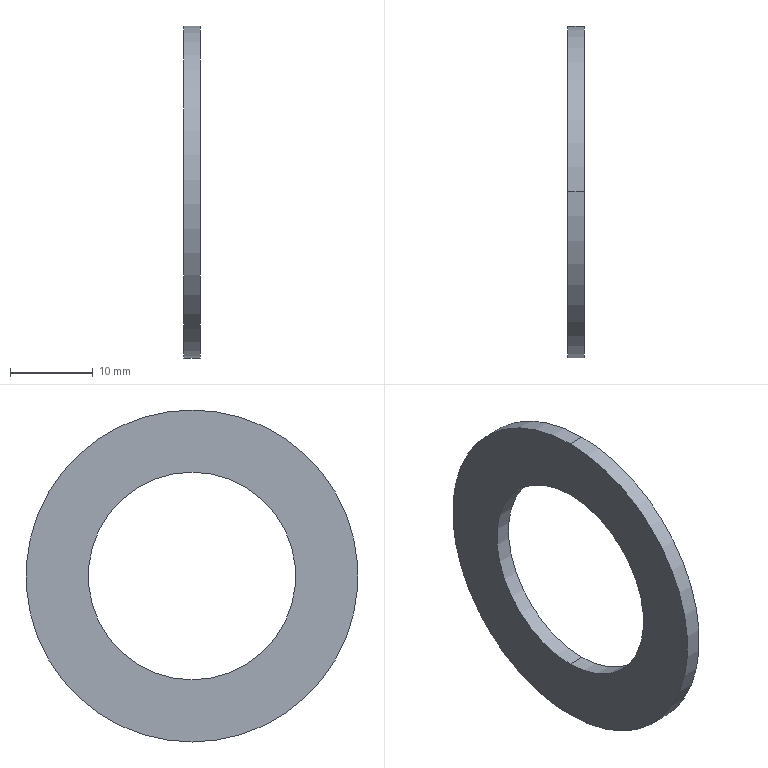Component | SolidWorks | 4-12-12ClampingAxisAssembly-1_4-12-8ClampingAxis51205BearingShim-1 | 1 solid | 6 faces | box 2 x 40 x 40 mm | volume 1532 mm3 | cylinder 4 | plane 2 | commonest cylinder face diameters 25 x2 40 x2
build123d program:
from build123d import *

# Parameters (mm, degrees)
SKETCH1_R      = 20
SKETCH1_R_2    = 12.5
EXTRUDE1_DEPTH = 2


with BuildPart() as part:
    # Sketch1 → Extrude1 (new body)
    with BuildSketch(Plane(origin=(0, 0, 0), x_dir=(1, 0, 0), z_dir=(0, 1, 0))):
        with Locations(Location((0, 0, 0), (0, 0, 270))):
            Circle(SKETCH1_R)
        with Locations(Location((0, 0, 0), (0, 0, 270))):
            Circle(SKETCH1_R_2, mode=Mode.SUBTRACT)
    extrude(amount=EXTRUDE1_DEPTH)


solid = part.part

# Placed as in the assembly
solid = solid.moved(Location((-53.809, -4.181, 0), (0, 0, 90)))
STEP:
#1=CARTESIAN_POINT('',(-2.197,-0.1646,-0.4921));
#2=VERTEX_POINT('',#1);
#3=CARTESIAN_POINT('',(-2.197,-0.1646,0.4921));
#4=VERTEX_POINT('',#3);
#5=CARTESIAN_POINT('',(-2.197,-0.1646,0.));
#6=DIRECTION('',(-1.,-0.,-0.));
#7=DIRECTION('',(0.,0.,1.));
#8=AXIS2_PLACEMENT_3D('',#5,#6,#7);
#9=CIRCLE('',#8,0.4921);
#10=EDGE_CURVE('',#2,#4,#9,.T.);
#11=ORIENTED_EDGE('',*,*,#10,.T.);
#12=CARTESIAN_POINT('',(-2.118,-0.1646,0.4921));
#13=VERTEX_POINT('',#12);
#14=CARTESIAN_POINT('',(-2.197,-0.1646,0.4921));
#15=DIRECTION('',(1.,0.,0.));
#16=VECTOR('',#15,39.37);
#17=LINE('',#14,#16);
#18=EDGE_CURVE('',#4,#13,#17,.T.);
#19=ORIENTED_EDGE('',*,*,#18,.T.);
#20=CARTESIAN_POINT('',(-2.118,-0.1646,-0.4921));
#21=VERTEX_POINT('',#20);
#22=CARTESIAN_POINT('',(-2.118,-0.1646,0.));
#23=DIRECTION('',(-1.,-0.,-0.));
#24=DIRECTION('',(0.,0.,1.));
#25=AXIS2_PLACEMENT_3D('',#22,#23,#24);
#26=CIRCLE('',#25,0.4921);
#27=EDGE_CURVE('',#21,#13,#26,.T.);
#28=ORIENTED_EDGE('',*,*,#27,.F.);
#29=CARTESIAN_POINT('',(-2.197,-0.1646,-0.4921));
#30=DIRECTION('',(1.,0.,0.));
#31=VECTOR('',#30,39.37);
#32=LINE('',#29,#31);
#33=EDGE_CURVE('',#2,#21,#32,.T.);
#34=ORIENTED_EDGE('',*,*,#33,.F.);
#35=EDGE_LOOP('',(#11,#19,#28,#34));
#36=FACE_OUTER_BOUND('',#35,.T.);
#37=CARTESIAN_POINT('',(-2.197,-0.1646,0.));
#38=DIRECTION('',(1.,0.,0.));
#39=DIRECTION('',(0.,-0.,-1.));
#40=AXIS2_PLACEMENT_3D('',#37,#38,#39);
#41=CYLINDRICAL_SURFACE('',#40,0.4921);
#42=ADVANCED_FACE('',(#36),#41,.F.);
#43=CARTESIAN_POINT('',(-2.197,-0.1646,0.7874));
#44=VERTEX_POINT('',#43);
#45=CARTESIAN_POINT('',(-2.197,-0.1646,-0.7874));
#46=VERTEX_POINT('',#45);
#47=CARTESIAN_POINT('',(-2.197,-0.1646,0.));
#48=DIRECTION('',(-1.,-0.,-0.));
#49=DIRECTION('',(0.,0.,1.));
#50=AXIS2_PLACEMENT_3D('',#47,#48,#49);
#51=CIRCLE('',#50,0.7874);
#52=EDGE_CURVE('',#44,#46,#51,.T.);
#53=ORIENTED_EDGE('',*,*,#52,.F.);
#54=CARTESIAN_POINT('',(-2.118,-0.1646,0.7874));
#55=VERTEX_POINT('',#54);
#56=CARTESIAN_POINT('',(-2.197,-0.1646,0.7874));
#57=DIRECTION('',(1.,0.,0.));
#58=VECTOR('',#57,39.37);
#59=LINE('',#56,#58);
#60=EDGE_CURVE('',#44,#55,#59,.T.);
#61=ORIENTED_EDGE('',*,*,#60,.T.);
#62=CARTESIAN_POINT('',(-2.118,-0.1646,-0.7874));
#63=VERTEX_POINT('',#62);
#64=CARTESIAN_POINT('',(-2.118,-0.1646,0.));
#65=DIRECTION('',(-1.,-0.,-0.));
#66=DIRECTION('',(0.,0.,1.));
#67=AXIS2_PLACEMENT_3D('',#64,#65,#66);
#68=CIRCLE('',#67,0.7874);
#69=EDGE_CURVE('',#55,#63,#68,.T.);
#70=ORIENTED_EDGE('',*,*,#69,.T.);
#71=CARTESIAN_POINT('',(-2.197,-0.1646,-0.7874));
#72=DIRECTION('',(1.,0.,0.));
#73=VECTOR('',#72,39.37);
#74=LINE('',#71,#73);
#75=EDGE_CURVE('',#46,#63,#74,.T.);
#76=ORIENTED_EDGE('',*,*,#75,.F.);
#77=EDGE_LOOP('',(#53,#61,#70,#76));
#78=FACE_OUTER_BOUND('',#77,.T.);
#79=CARTESIAN_POINT('',(-2.197,-0.1646,0.));
#80=DIRECTION('',(1.,0.,0.));
#81=DIRECTION('',(0.,-0.,-1.));
#82=AXIS2_PLACEMENT_3D('',#79,#80,#81);
#83=CYLINDRICAL_SURFACE('',#82,0.7874);
#84=ADVANCED_FACE('',(#78),#83,.T.);
#85=CARTESIAN_POINT('',(-2.197,-0.1646,0.));
#86=DIRECTION('',(-1.,-0.,-0.));
#87=DIRECTION('',(0.,0.,1.));
#88=AXIS2_PLACEMENT_3D('',#85,#86,#87);
#89=CIRCLE('',#88,0.7874);
#90=EDGE_CURVE('',#46,#44,#89,.T.);
#91=ORIENTED_EDGE('',*,*,#90,.T.);
#92=ORIENTED_EDGE('',*,*,#52,.T.);
#93=EDGE_LOOP('',(#91,#92));
#94=FACE_OUTER_BOUND('',#93,.T.);
#95=ORIENTED_EDGE('',*,*,#10,.F.);
#96=CARTESIAN_POINT('',(-2.197,-0.1646,0.));
#97=DIRECTION('',(-1.,-0.,-0.));
#98=DIRECTION('',(0.,0.,1.));
#99=AXIS2_PLACEMENT_3D('',#96,#97,#98);
#100=CIRCLE('',#99,0.4921);
#101=EDGE_CURVE('',#4,#2,#100,.T.);
#102=ORIENTED_EDGE('',*,*,#101,.F.);
#103=EDGE_LOOP('',(#95,#102));
#104=FACE_BOUND('',#103,.T.);
#105=CARTESIAN_POINT('',(-2.197,-0.1646,0.));
#106=DIRECTION('',(-1.,-0.,-0.));
#107=DIRECTION('',(-0.,0.,1.));
#108=AXIS2_PLACEMENT_3D('',#105,#106,#107);
#109=PLANE('',#108);
#110=ADVANCED_FACE('',(#94,#104),#109,.T.);
#111=CARTESIAN_POINT('',(-2.118,-0.1646,0.));
#112=DIRECTION('',(-1.,-0.,-0.));
#113=DIRECTION('',(0.,0.,1.));
#114=AXIS2_PLACEMENT_3D('',#111,#112,#113);
#115=CIRCLE('',#114,0.7874);
#116=EDGE_CURVE('',#63,#55,#115,.T.);
#117=ORIENTED_EDGE('',*,*,#116,.F.);
#118=ORIENTED_EDGE('',*,*,#69,.F.);
#119=EDGE_LOOP('',(#117,#118));
#120=FACE_OUTER_BOUND('',#119,.T.);
#121=ORIENTED_EDGE('',*,*,#27,.T.);
#122=CARTESIAN_POINT('',(-2.118,-0.1646,0.));
#123=DIRECTION('',(-1.,-0.,-0.));
#124=DIRECTION('',(0.,0.,1.));
#125=AXIS2_PLACEMENT_3D('',#122,#123,#124);
#126=CIRCLE('',#125,0.4921);
#127=EDGE_CURVE('',#13,#21,#126,.T.);
#128=ORIENTED_EDGE('',*,*,#127,.T.);
#129=EDGE_LOOP('',(#121,#128));
#130=FACE_BOUND('',#129,.T.);
#131=CARTESIAN_POINT('',(-2.118,-0.1646,0.));
#132=DIRECTION('',(-1.,-0.,-0.));
#133=DIRECTION('',(-0.,0.,1.));
#134=AXIS2_PLACEMENT_3D('',#131,#132,#133);
#135=PLANE('',#134);
#136=ADVANCED_FACE('',(#120,#130),#135,.F.);
#137=ORIENTED_EDGE('',*,*,#60,.F.);
#138=ORIENTED_EDGE('',*,*,#90,.F.);
#139=ORIENTED_EDGE('',*,*,#75,.T.);
#140=ORIENTED_EDGE('',*,*,#116,.T.);
#141=EDGE_LOOP('',(#137,#138,#139,#140));
#142=FACE_OUTER_BOUND('',#141,.T.);
#143=CARTESIAN_POINT('',(-2.197,-0.1646,0.));
#144=DIRECTION('',(1.,0.,0.));
#145=DIRECTION('',(0.,-0.,-1.));
#146=AXIS2_PLACEMENT_3D('',#143,#144,#145);
#147=CYLINDRICAL_SURFACE('',#146,0.7874);
#148=ADVANCED_FACE('',(#142),#147,.T.);
#149=ORIENTED_EDGE('',*,*,#18,.F.);
#150=ORIENTED_EDGE('',*,*,#101,.T.);
#151=ORIENTED_EDGE('',*,*,#33,.T.);
#152=ORIENTED_EDGE('',*,*,#127,.F.);
#153=EDGE_LOOP('',(#149,#150,#151,#152));
#154=FACE_OUTER_BOUND('',#153,.T.);
#155=CARTESIAN_POINT('',(-2.197,-0.1646,0.));
#156=DIRECTION('',(1.,0.,0.));
#157=DIRECTION('',(0.,-0.,-1.));
#158=AXIS2_PLACEMENT_3D('',#155,#156,#157);
#159=CYLINDRICAL_SURFACE('',#158,0.4921);
#160=ADVANCED_FACE('',(#154),#159,.F.);
#161=CLOSED_SHELL('',(#42,#84,#110,#136,#148,#160));
#162=MANIFOLD_SOLID_BREP('',#161);
#163=CARTESIAN_POINT('',(0.,0.,0.));
#164=DIRECTION('',(0.,0.,1.));
#165=DIRECTION('',(1.,0.,0.));
#166=AXIS2_PLACEMENT_3D('',#163,#164,#165);
#167=(LENGTH_UNIT()NAMED_UNIT(*)SI_UNIT($,.METRE.));
#168=LENGTH_MEASURE_WITH_UNIT(LENGTH_MEASURE(0.0254),#167);
#169=DIMENSIONAL_EXPONENTS(1.,0.,0.,0.,0.,0.,0.);
#170=(CONVERSION_BASED_UNIT('',#168)LENGTH_UNIT()NAMED_UNIT(#169));
#171=UNCERTAINTY_MEASURE_WITH_UNIT(LENGTH_MEASURE(0.00001),#170,'','');
#172=(NAMED_UNIT(*)PLANE_ANGLE_UNIT()SI_UNIT($,.RADIAN.));
#173=(NAMED_UNIT(*)SI_UNIT($,.STERADIAN.)SOLID_ANGLE_UNIT());
#174=(GEOMETRIC_REPRESENTATION_CONTEXT(3)GLOBAL_UNCERTAINTY_ASSIGNED_CONTEXT((#171))GLOBAL_UNIT_ASSIGNED_CONTEXT((#170,#172,#173))REPRESENTATION_CONTEXT('',''));
#175=ADVANCED_BREP_SHAPE_REPRESENTATION('',(#162,#166),#174);
#176=COLOUR_RGB('',0.7922,0.8196,0.9333);
#177=FILL_AREA_STYLE_COLOUR('',#176);
#178=FILL_AREA_STYLE('',(#177));
#179=SURFACE_STYLE_FILL_AREA(#178);
#180=SURFACE_SIDE_STYLE('',(#179));
#181=SURFACE_STYLE_USAGE(.BOTH.,#180);
#182=PRESENTATION_STYLE_ASSIGNMENT((#181));
#183=STYLED_ITEM('',(#182),#162);
#184=(LENGTH_UNIT()NAMED_UNIT(*)SI_UNIT($,.METRE.));
#185=LENGTH_MEASURE_WITH_UNIT(LENGTH_MEASURE(0.0254),#184);
#186=DIMENSIONAL_EXPONENTS(1.,0.,0.,0.,0.,0.,0.);
#187=(CONVERSION_BASED_UNIT('',#185)LENGTH_UNIT()NAMED_UNIT(#186));
#188=UNCERTAINTY_MEASURE_WITH_UNIT(LENGTH_MEASURE(0.00001),#187,'','');
#189=(NAMED_UNIT(*)PLANE_ANGLE_UNIT()SI_UNIT($,.RADIAN.));
#190=(NAMED_UNIT(*)SI_UNIT($,.STERADIAN.)SOLID_ANGLE_UNIT());
#191=(GEOMETRIC_REPRESENTATION_CONTEXT(3)GLOBAL_UNCERTAINTY_ASSIGNED_CONTEXT((#188))GLOBAL_UNIT_ASSIGNED_CONTEXT((#187,#189,#190))REPRESENTATION_CONTEXT('',''));
#192=MECHANICAL_DESIGN_GEOMETRIC_PRESENTATION_REPRESENTATION('',(#183),#191);
#193=PRESENTATION_LAYER_ASSIGNMENT('','',(#183));